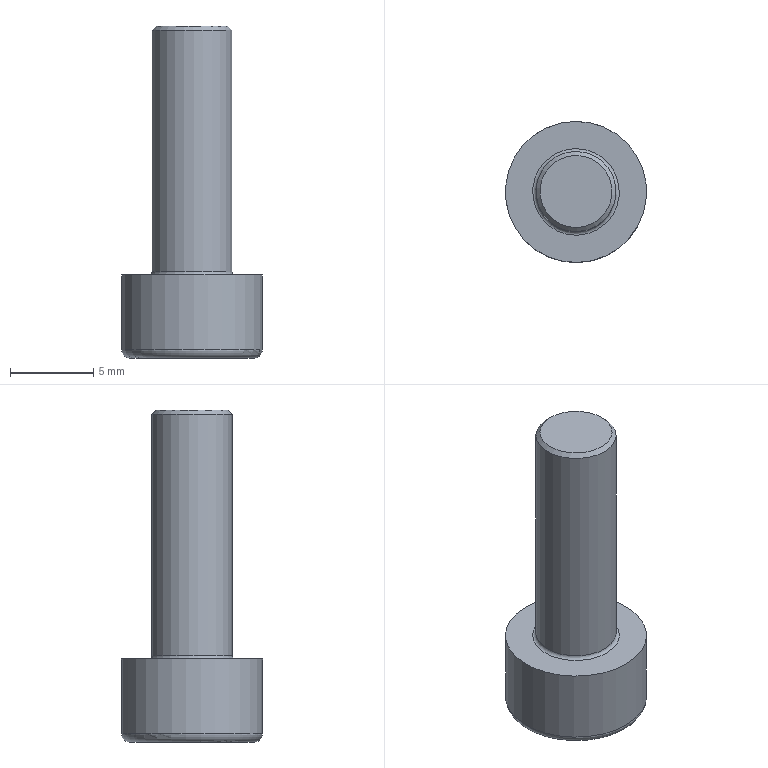Component | NX | GB-T70_1-2000_M5X15_2 | 1 solid | 27 faces | volume 508 mm3 | plane 15 | cone 8 | cylinder 2 | torus 2 | commonest cylinder face diameters 4.826 x1 8.5 x1